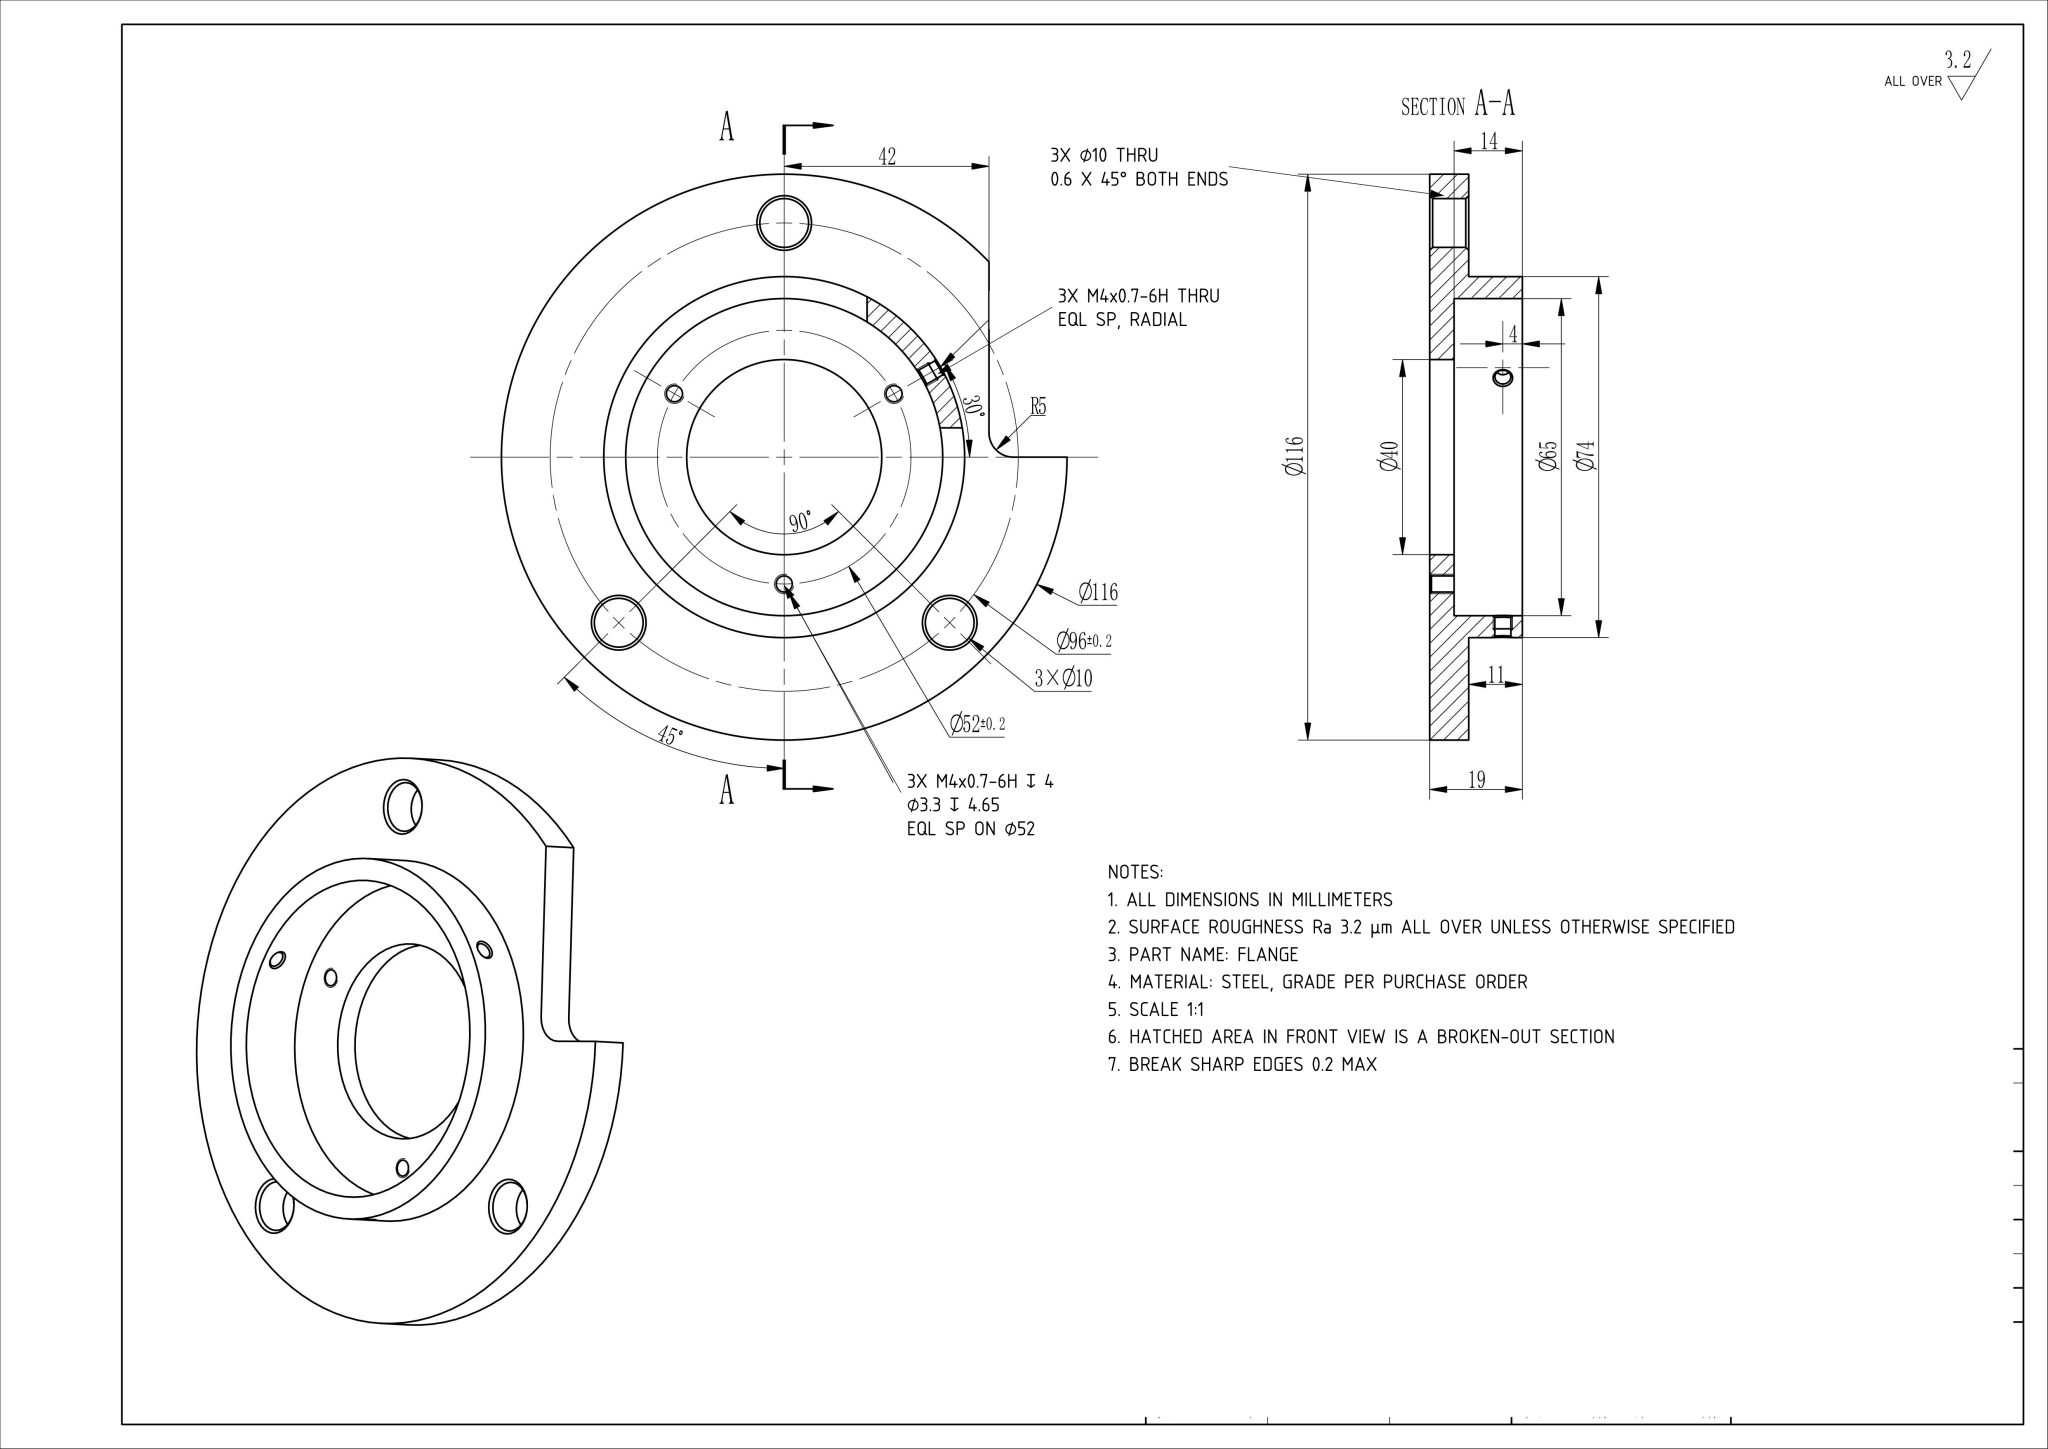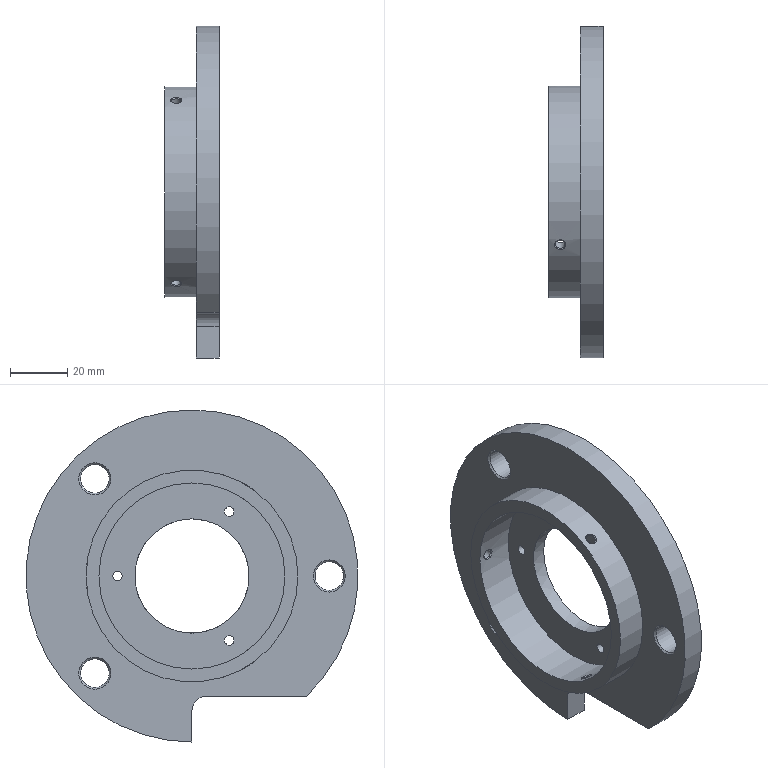Part | NX | mm | 1 solid | 35 faces | box 19 x 116 x 116 mm | volume 73470 mm3 | cylinder 14 | cone 9 | plane 6 | spline 6 | commonest cylinder face diameters 3.3 x6 10 x4 40 x1 116 x1 74 x1 65 x1